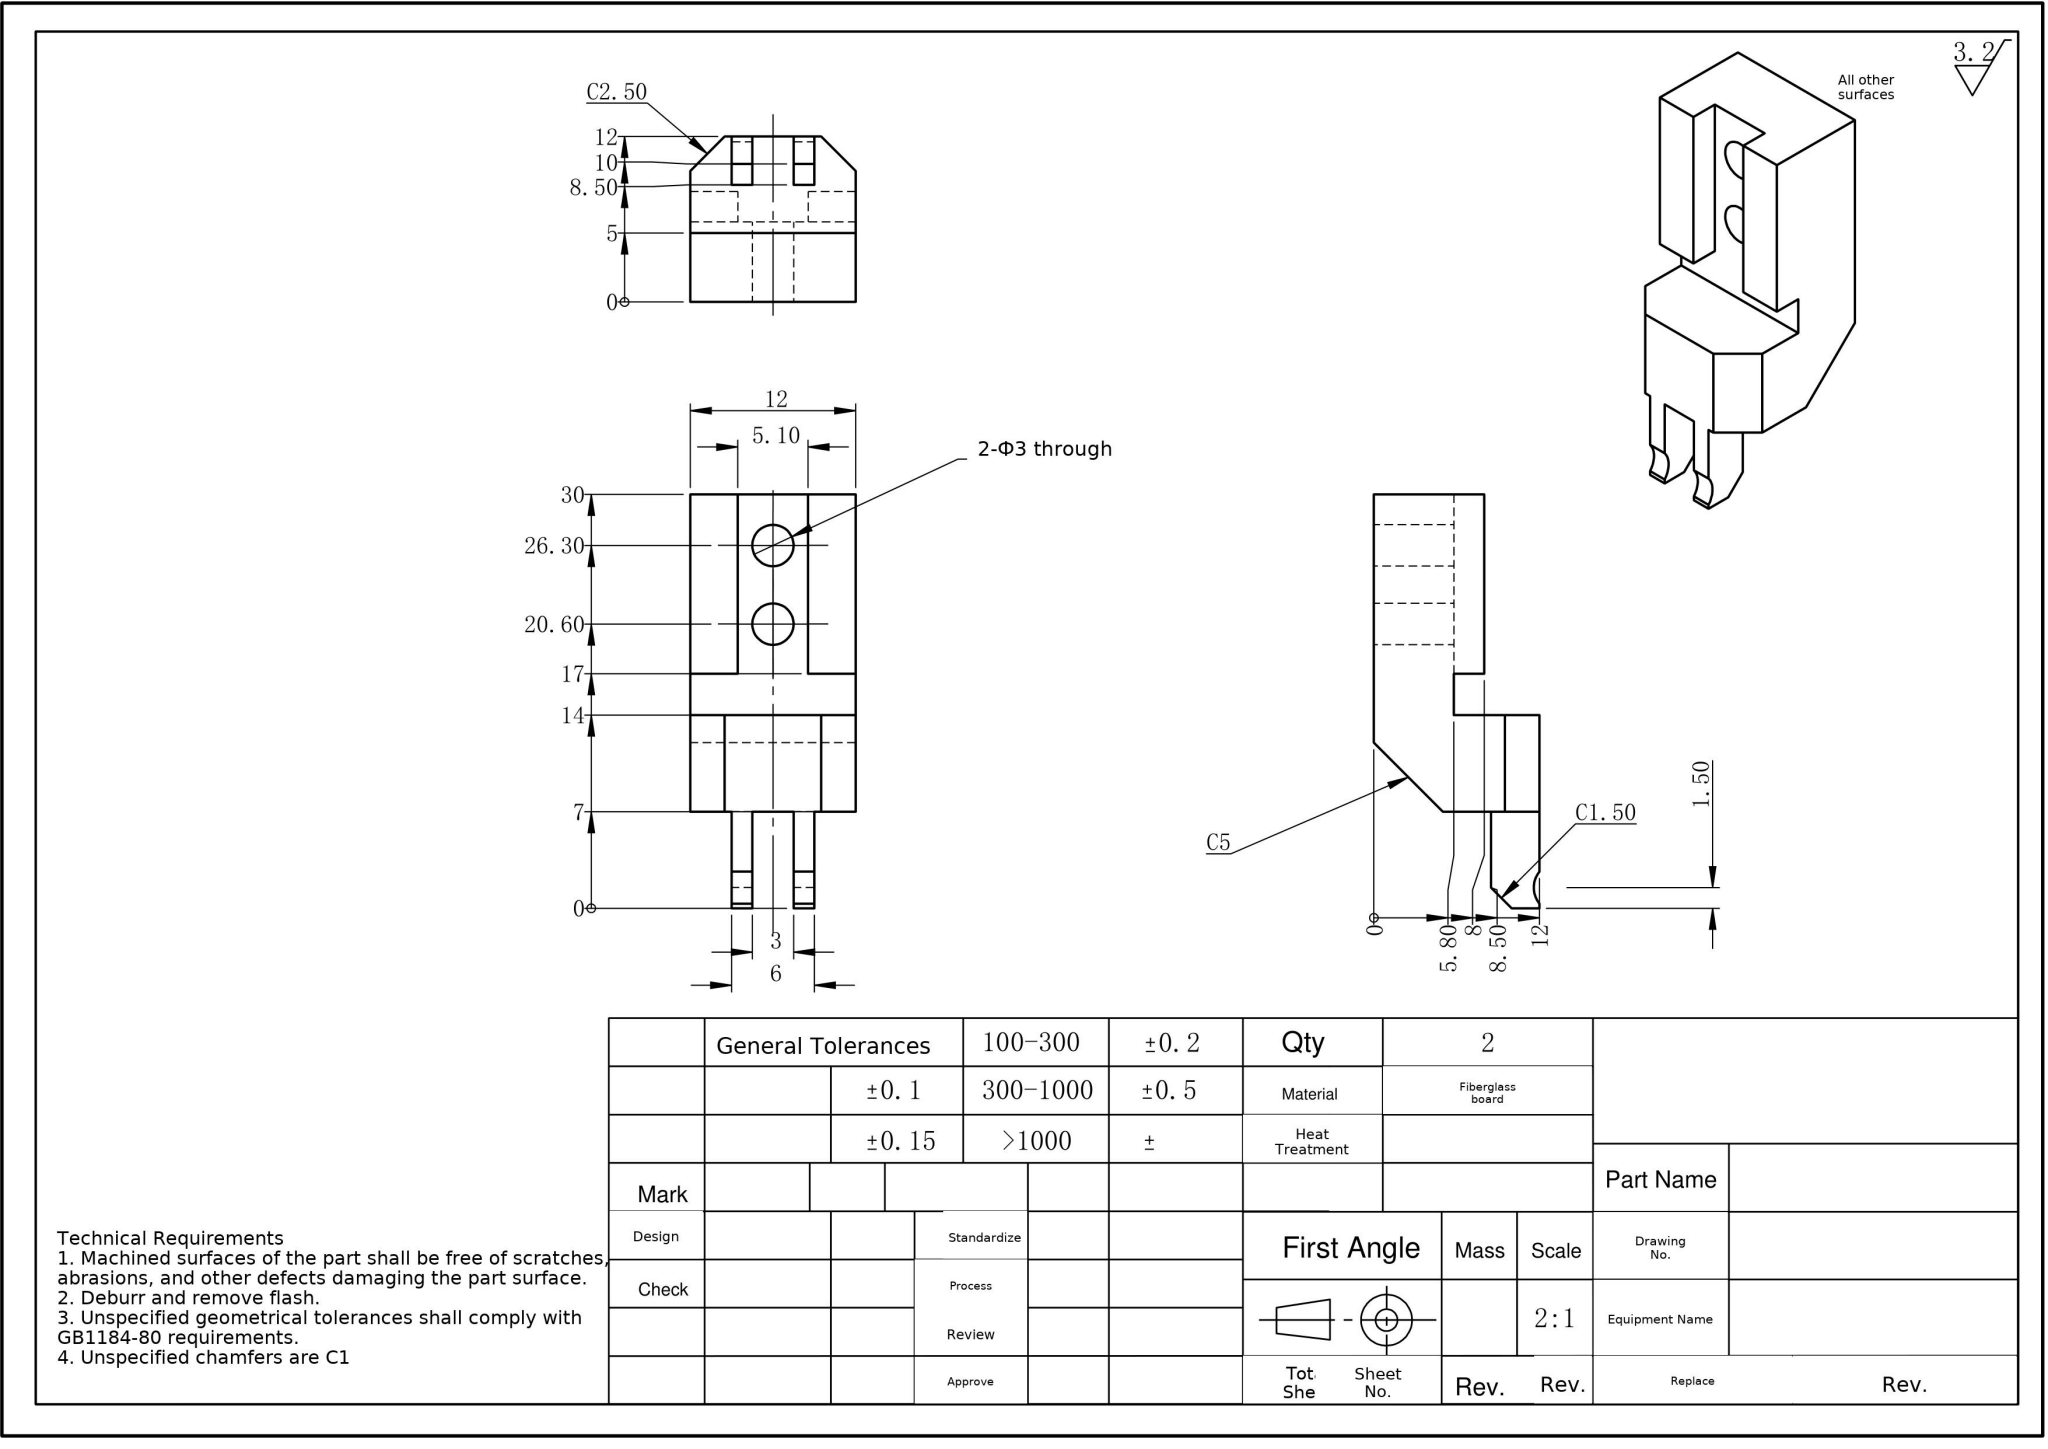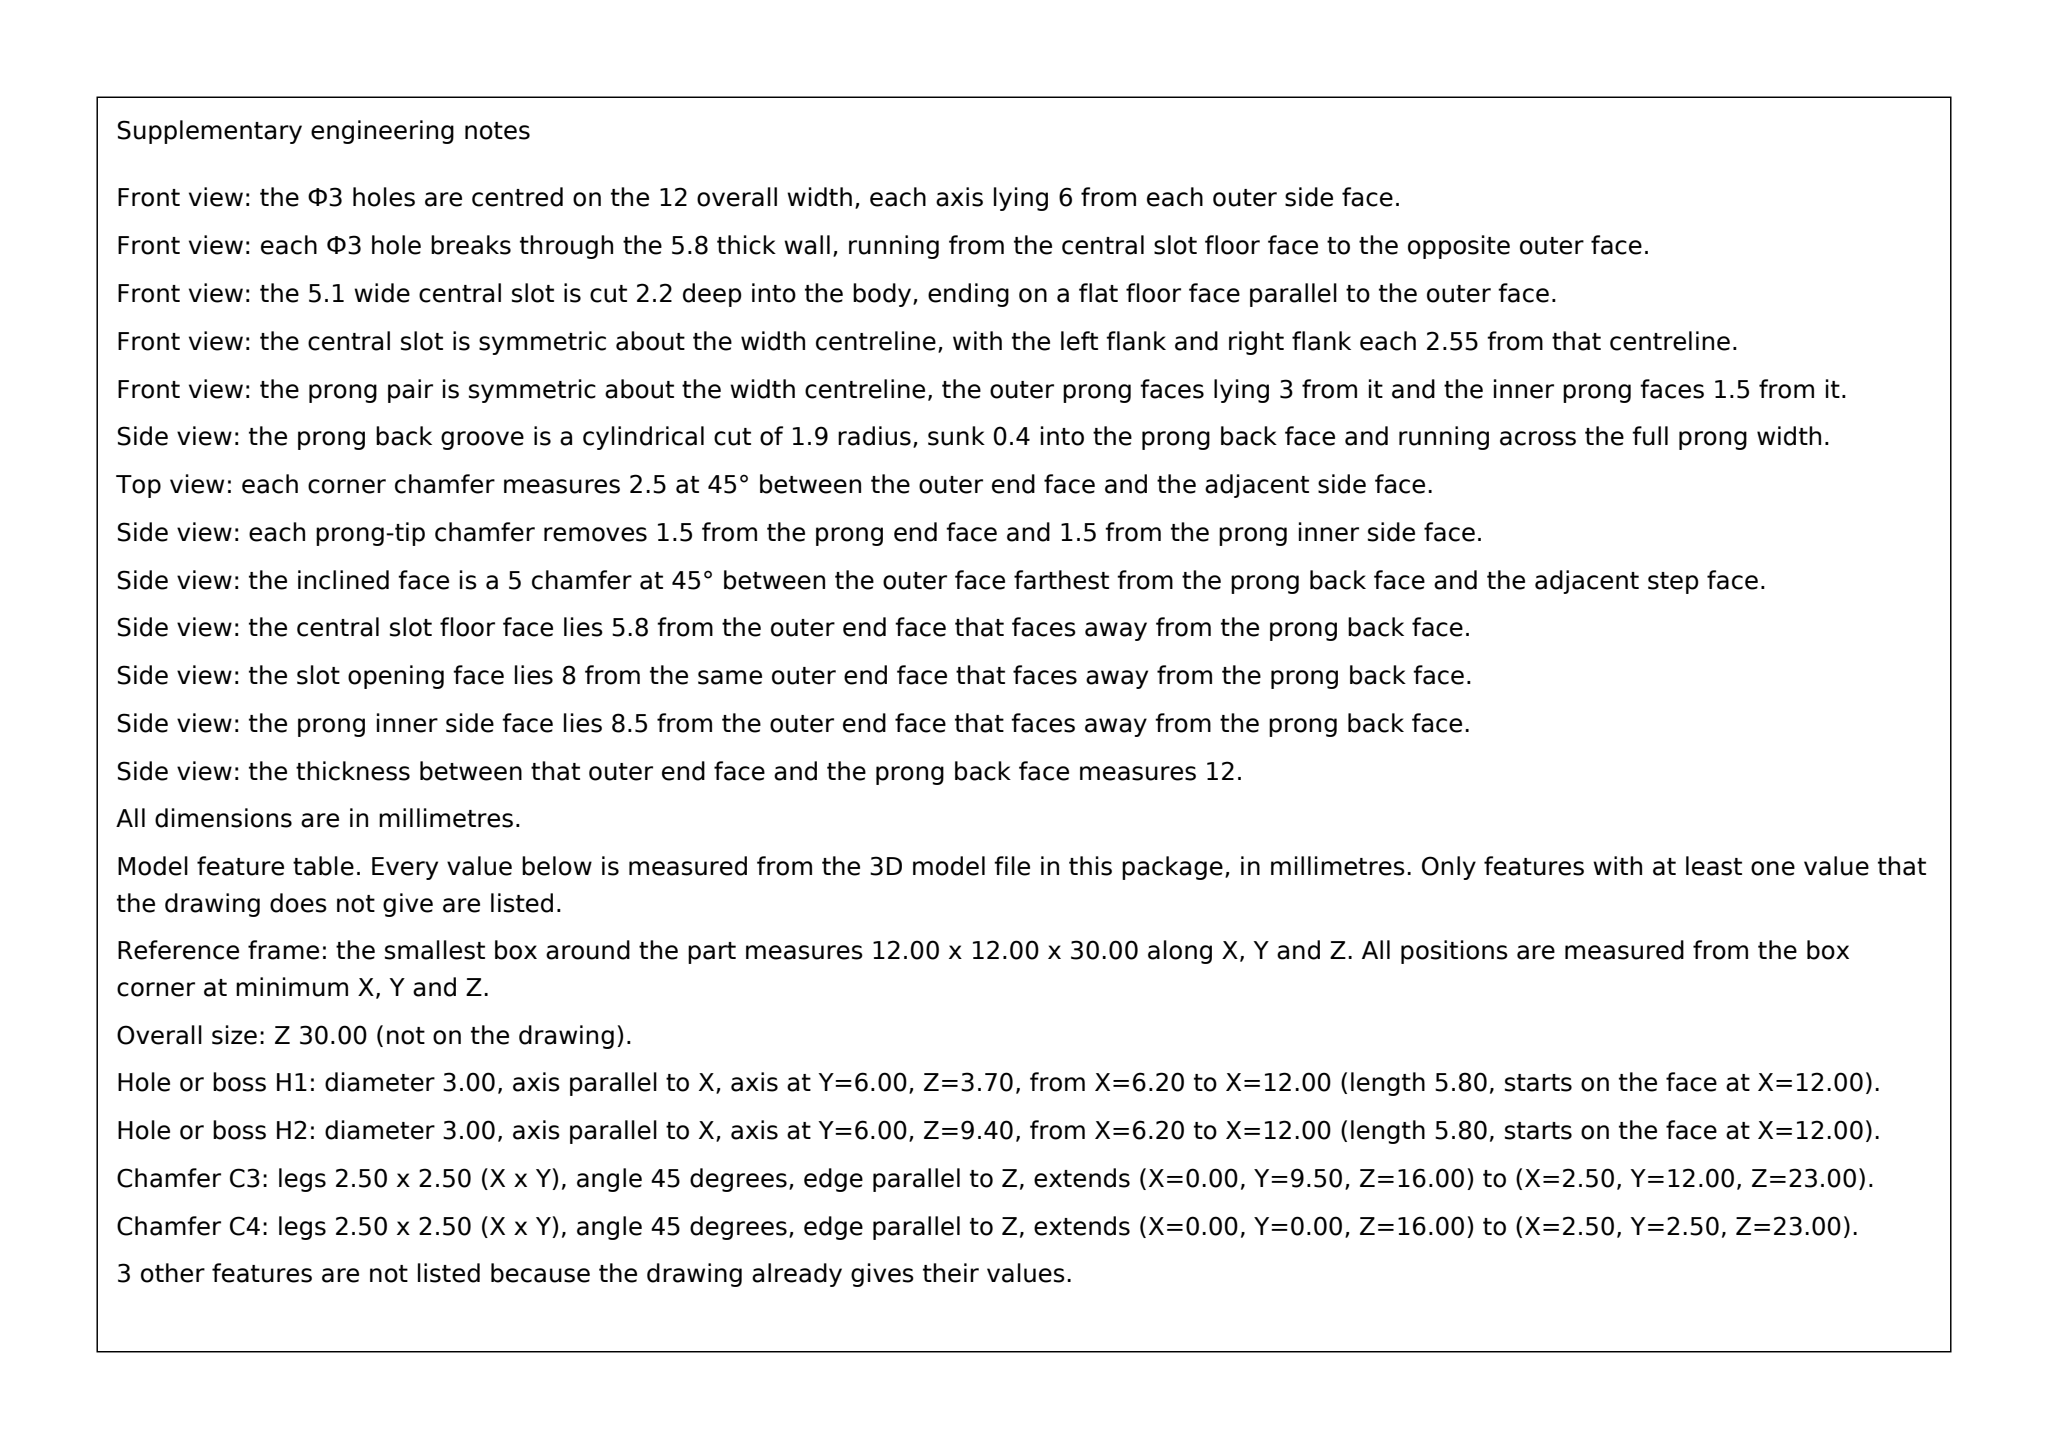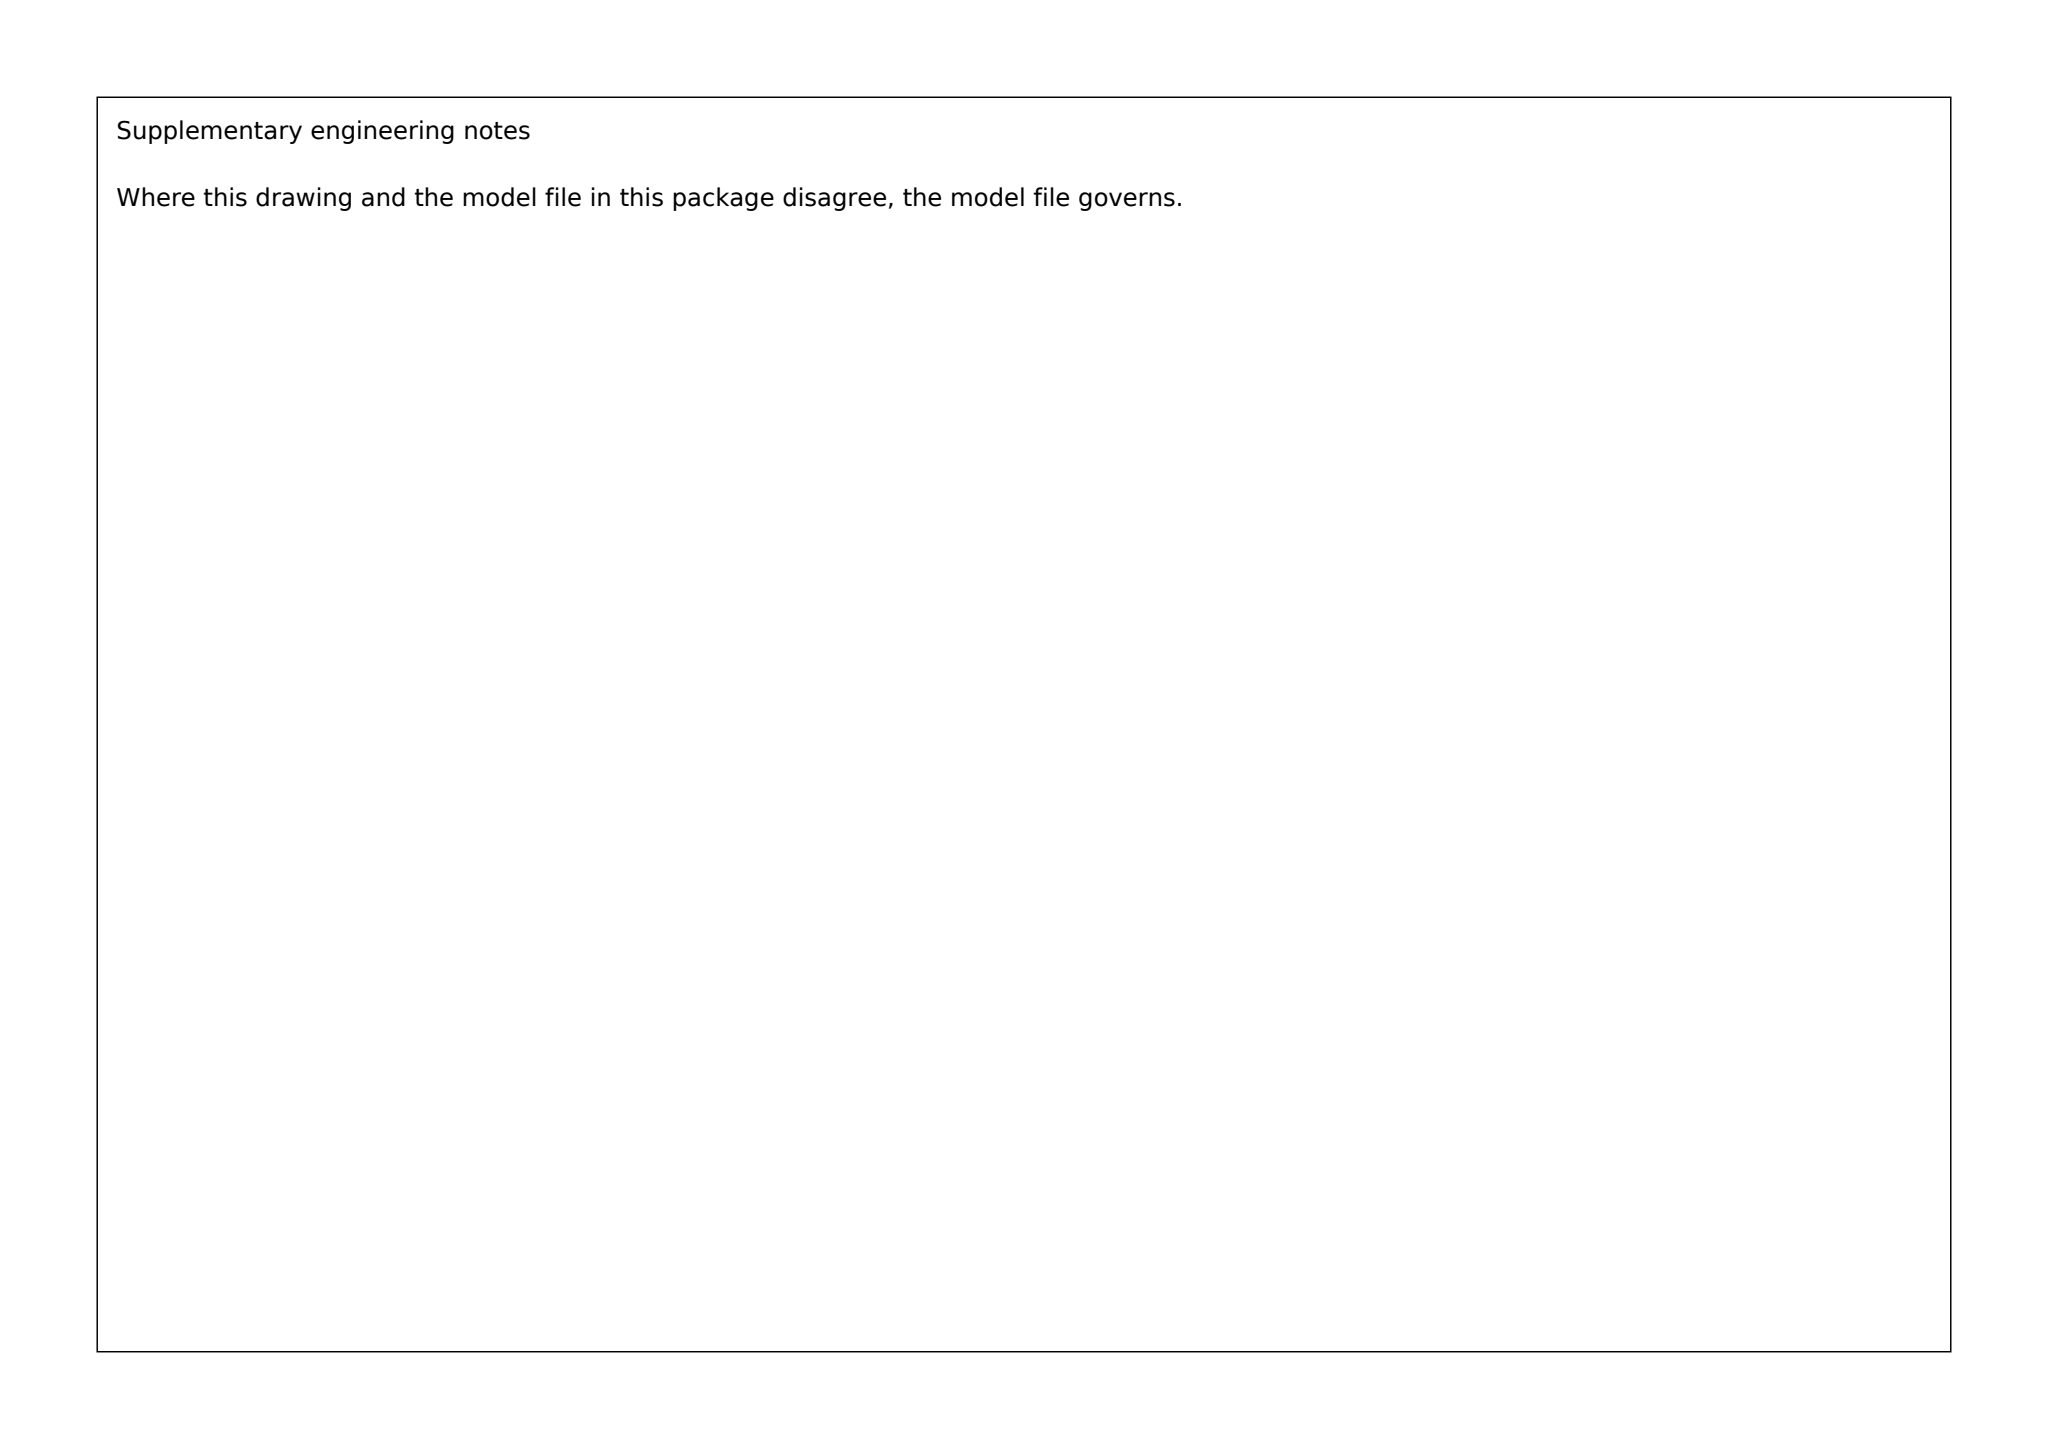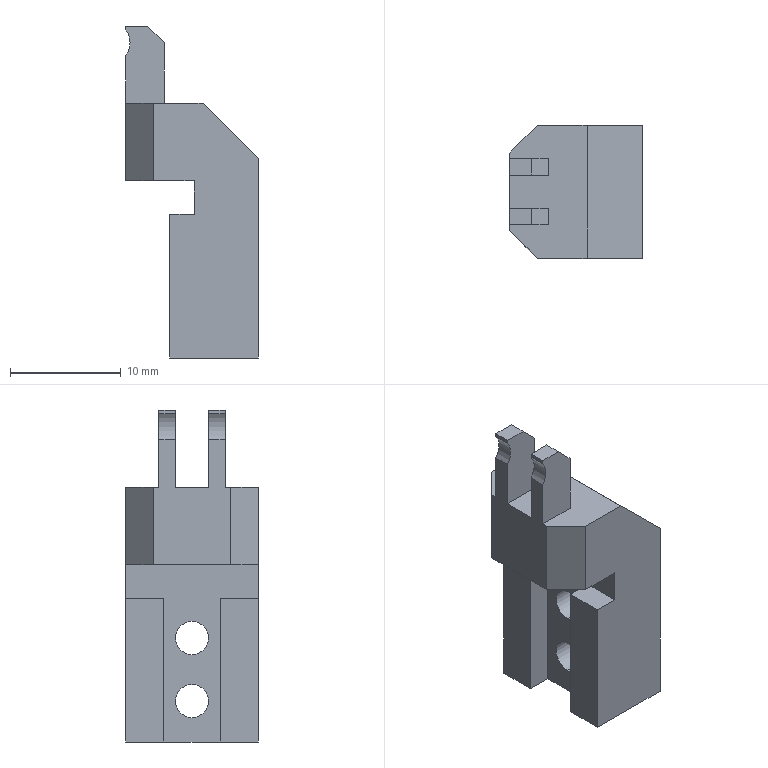Part | SolidWorks | mm | material Fiberglass board | 1 solid | 35 faces | box 12 x 12 x 30 mm | volume 2111 mm3 | plane 29 | cylinder 6 | commonest cylinder face diameters 3 x4 3.8 x2
Drawing notes:
2X R1.90 NOTCH AT PRONG TIP, CTR 1.50 FROM END & 1.50 OFF FACE | from the solid: cylinders: [3.8 dia, axis y, pos x=-1.5, z=28.5, len 1.5, count 2]; R=1.9, axis 1.5 beyond x=0 face and 1.5 from z=30 end (drawing 0 datum)
NOTCH 0.40 DP INTO 12 FACE, FULL 1.50 PRONG THK, 2X | from the solid: R1.9 cyl ctr 1.5 outside side face: 1.9-1.5=0.40 cut depth; cyl length 1.5 = prong thk (y planes 3.0/4.5 and 7.5/9.0)
DISREGARD C1.50: PRONG TIP CORNER IS R1.90 x 0.40 DP | from the solid: no chamfer face at that corner in STEP; only 3.8 dia (R1.90) cylinder, axis y, pos x=-1.5, z=28.5, len 1.5